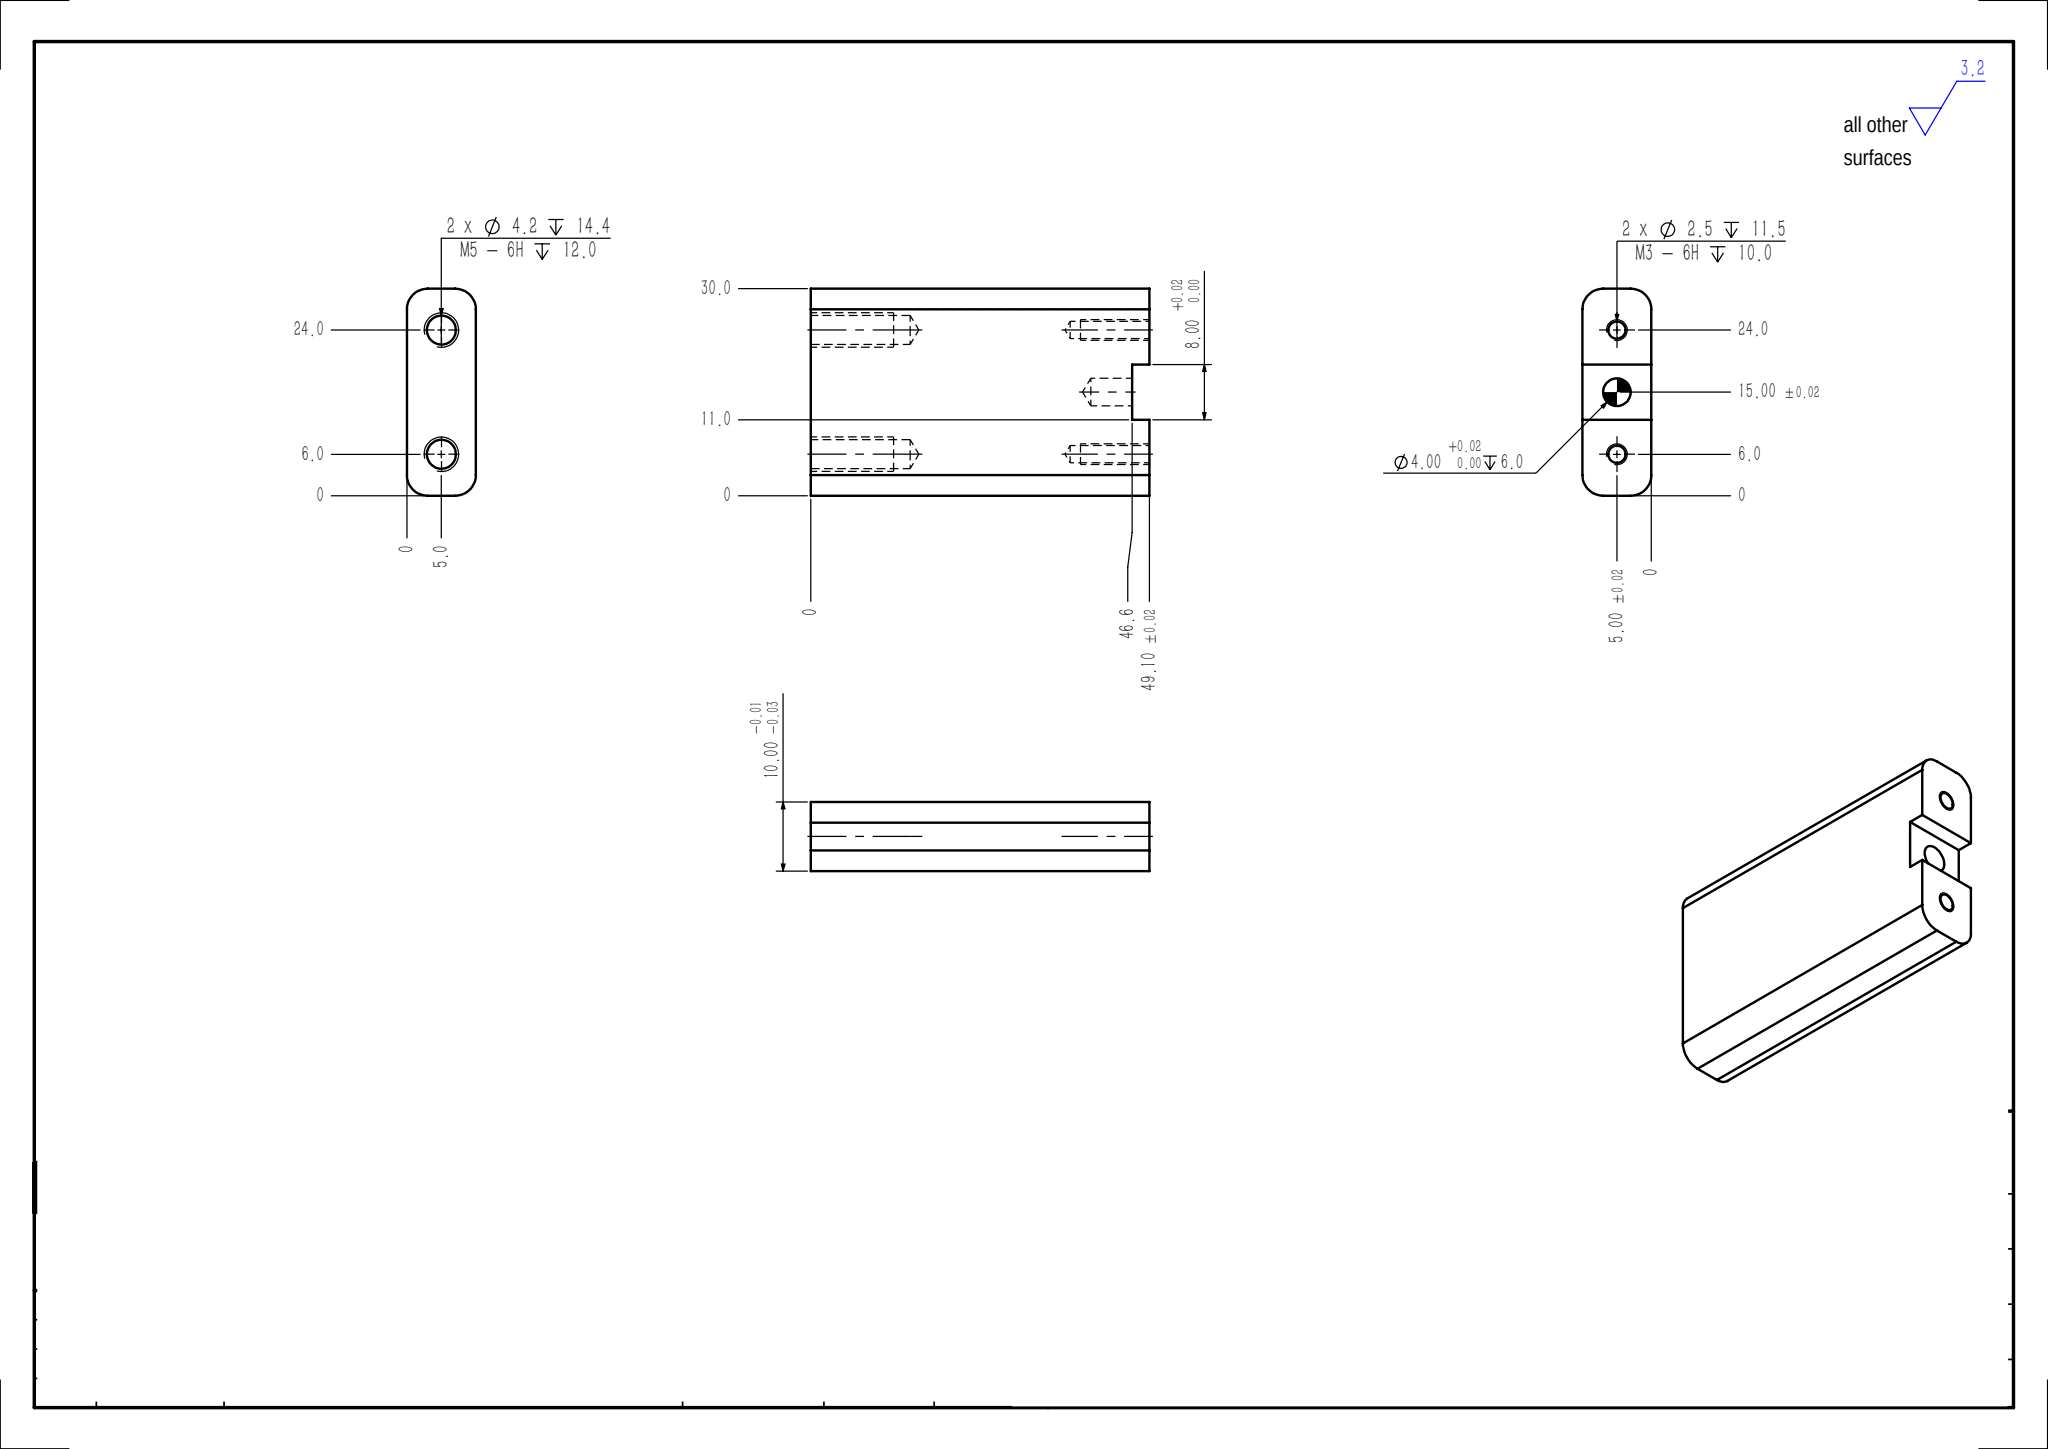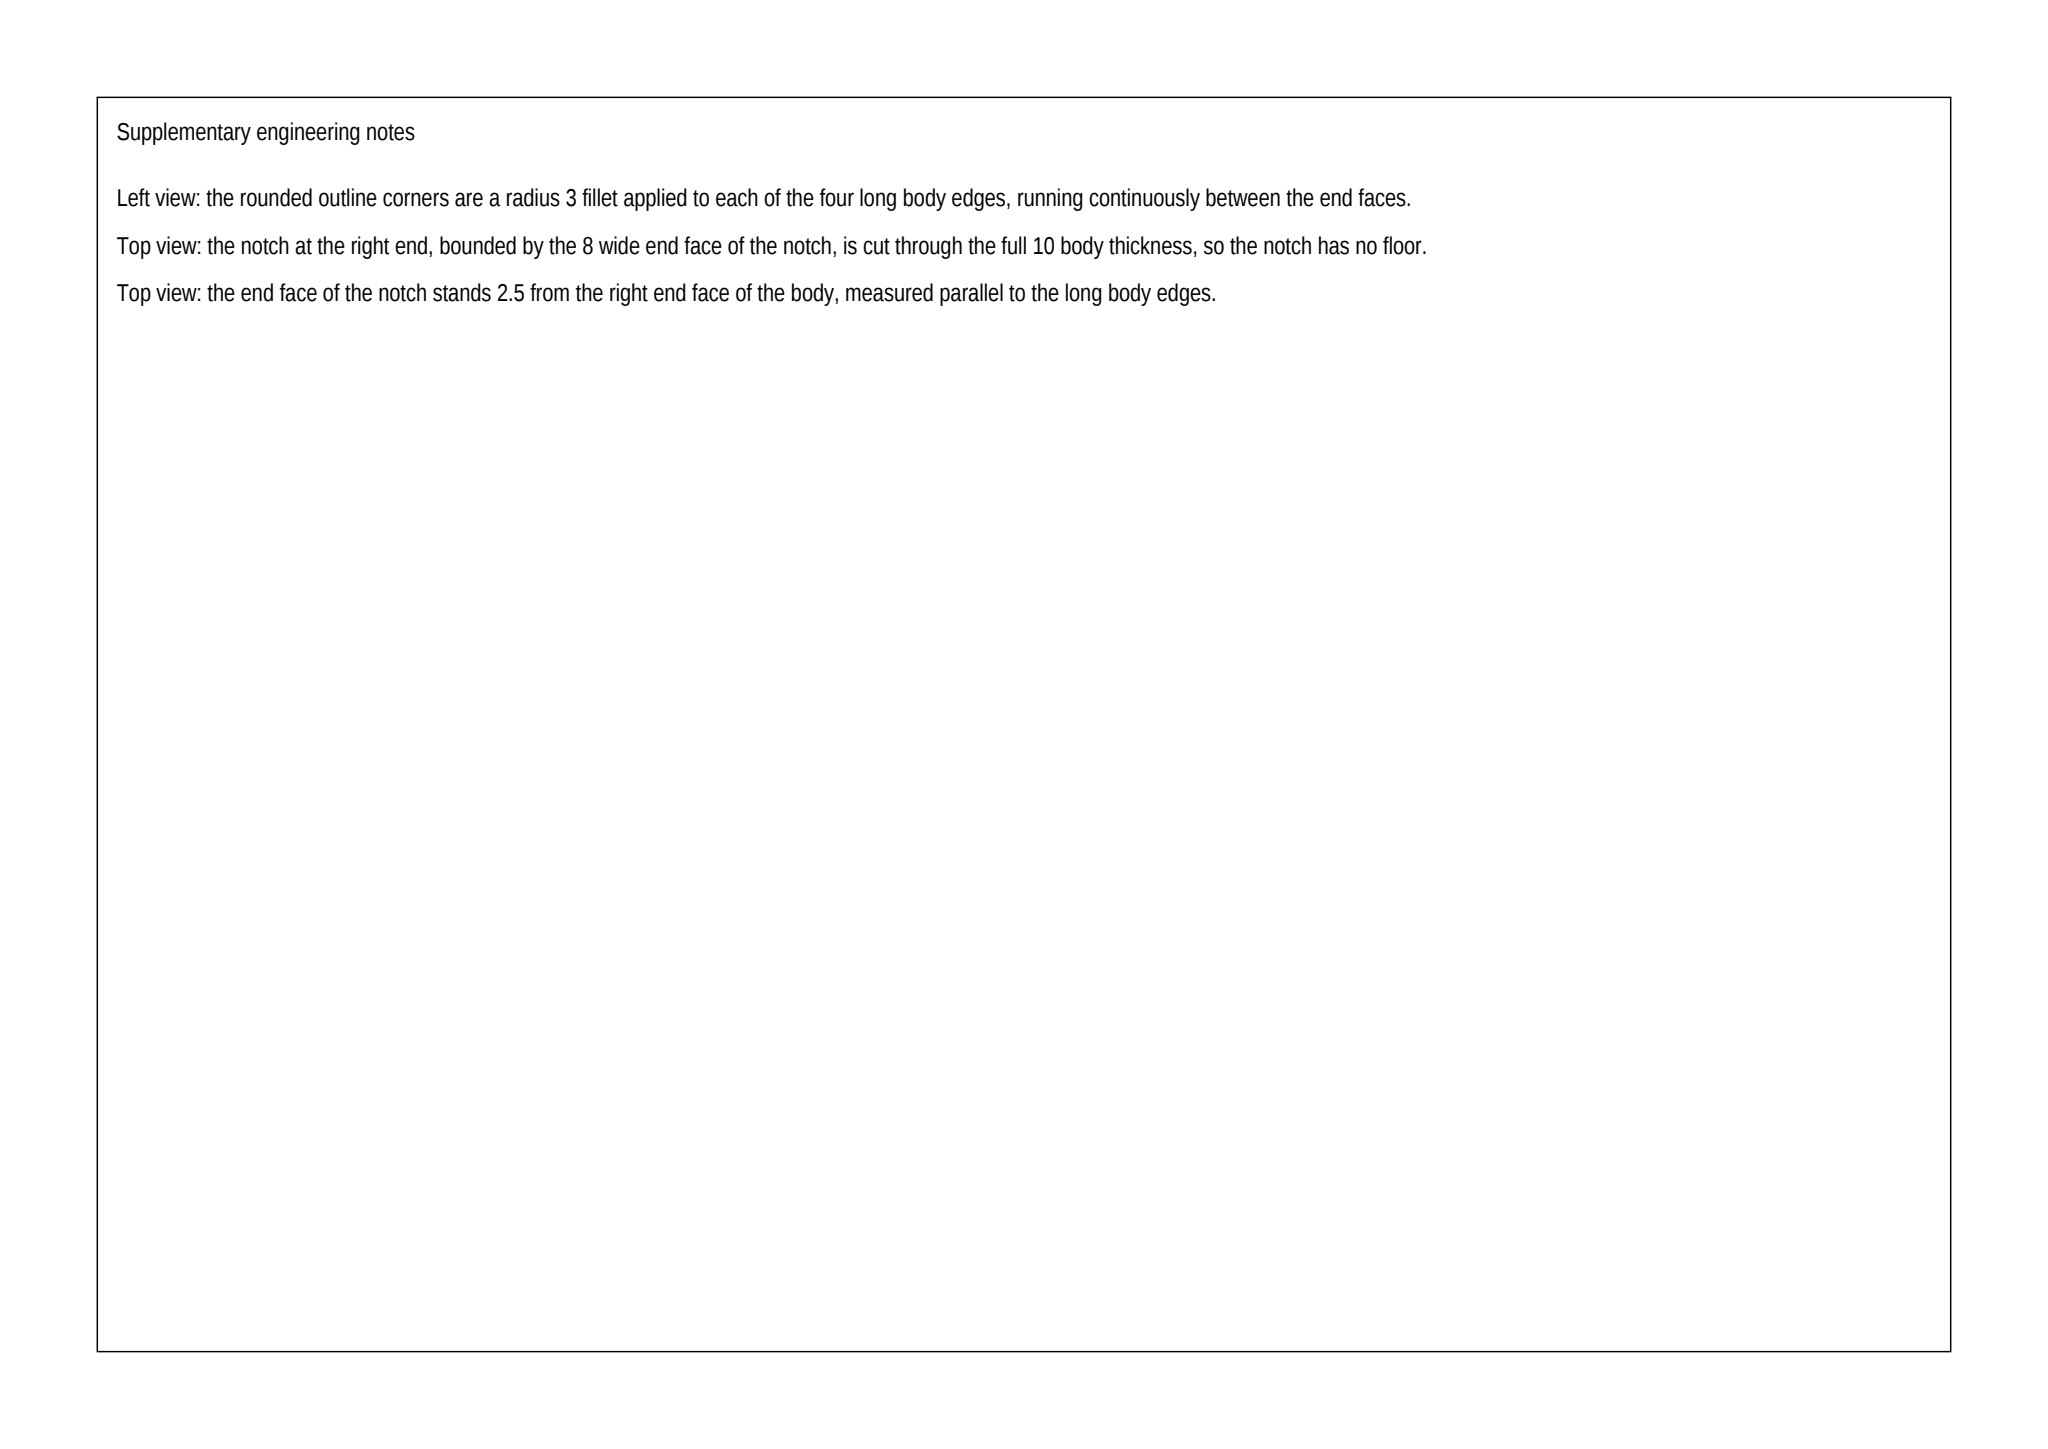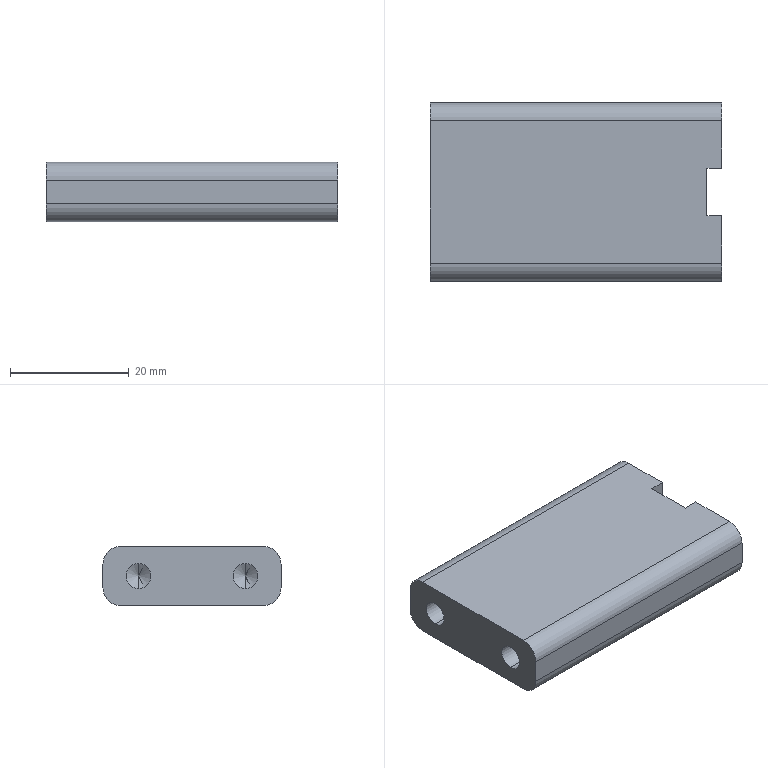Part | SolidWorks | mm | 1 solid | 34 faces | box 49.1 x 30 x 10 mm | volume 13544 mm3 | cylinder 14 | cone 10 | plane 10 | commonest cylinder face diameters 2.5 x4 4.2 x4 6 x4 4 x2
Drawing notes:
4X R3 ROUND ON LONG EDGES, FULL LENGTH 49.10 | from the solid: Four Ø6 cylinders, axis x, len 49.1, at (y,z)=(3,3),(3,7),(27,3),(27,7) => R3 at bar corners
build123d program:
from build123d import *

# Parameters (mm, degrees)
SKETCH1_W                      = 49.1
SKETCH1_H                      = 30
BOSS_EXTRUDE1_DEPTH            = 5
M5_TAPPED_HOLE1_D              = 4.2
M5_TAPPED_HOLE1_DEPTH          = 14.4
M5_TAPPED_HOLE1_TIP            = 1.262
FILLET1_R                      = 3
SKETCH6_W                      = 10
SKETCH6_H                      = 8
CUT_EXTRUDE2_DEPTH             = 2.5
M3_TAPPED_HOLE1_D              = 2.5
M3_TAPPED_HOLE1_DEPTH          = 11.5
M3_TAPPED_HOLE1_TIP            = 0.7511
SIZE_MM_DOWEL_PIN_HOLE_1_D     = 4
SIZE_MM_DOWEL_PIN_HOLE_1_DEPTH = 6
SIZE_MM_DOWEL_PIN_HOLE_1_TIP   = 1.202


with BuildPart() as part:
    # Sketch1 → Boss-Extrude1 (new, symmetric)
    with BuildSketch(Plane.XY):
        Rectangle(SKETCH1_W, SKETCH1_H)
    extrude(amount=BOSS_EXTRUDE1_DEPTH, both=True)

    # M5 Tapped Hole1
    with Locations(Plane.ZY.offset(24.55)):
        with Locations((0, 9), (0, -9)):
            Hole(M5_TAPPED_HOLE1_D / 2, depth=M5_TAPPED_HOLE1_DEPTH)
            with Locations((0, 0, -(M5_TAPPED_HOLE1_DEPTH + M5_TAPPED_HOLE1_TIP / 2))):  # 118° drill point
                Cone(0, M5_TAPPED_HOLE1_D / 2, M5_TAPPED_HOLE1_TIP, mode=Mode.SUBTRACT)

    # Fillet1
    fillet1_edges = [part.edges().sort_by_distance(p)[0] for p in [
        (0, -15, 5),
        (0, -15, -5),
        (0, 15, -5),
        (0, 15, 5),
    ]]
    fillet(fillet1_edges, radius=FILLET1_R)

    # Sketch6 → Cut-Extrude2 (cut)
    with BuildSketch(Plane(origin=(24.55, 0, 0), x_dir=(0, 0, -1), z_dir=(1, 0, 0))):
        Rectangle(SKETCH6_W, SKETCH6_H)
    extrude(amount=-CUT_EXTRUDE2_DEPTH, mode=Mode.SUBTRACT)

    # M3 Tapped Hole1
    with Locations(Plane(origin=(24.55, 0, 0), x_dir=(0, 0, -1), z_dir=(1, 0, 0))):
        with Locations((0, 9), (0, -9)):
            Hole(M3_TAPPED_HOLE1_D / 2, depth=M3_TAPPED_HOLE1_DEPTH)
            with Locations((0, 0, -(M3_TAPPED_HOLE1_DEPTH + M3_TAPPED_HOLE1_TIP / 2))):  # 118° drill point
                Cone(0, M3_TAPPED_HOLE1_D / 2, M3_TAPPED_HOLE1_TIP, mode=Mode.SUBTRACT)

    # Size mm Dowel Pin Hole 1
    with Locations(Plane(origin=(22.05, 0, 0), x_dir=(0, 0, -1), z_dir=(1, 0, 0))):
        with Locations((0, 0)):
            Hole(SIZE_MM_DOWEL_PIN_HOLE_1_D / 2, depth=SIZE_MM_DOWEL_PIN_HOLE_1_DEPTH)
            with Locations((0, 0, -(SIZE_MM_DOWEL_PIN_HOLE_1_DEPTH + SIZE_MM_DOWEL_PIN_HOLE_1_TIP / 2))):  # 118° drill point
                Cone(0, SIZE_MM_DOWEL_PIN_HOLE_1_D / 2, SIZE_MM_DOWEL_PIN_HOLE_1_TIP, mode=Mode.SUBTRACT)


solid = part.part